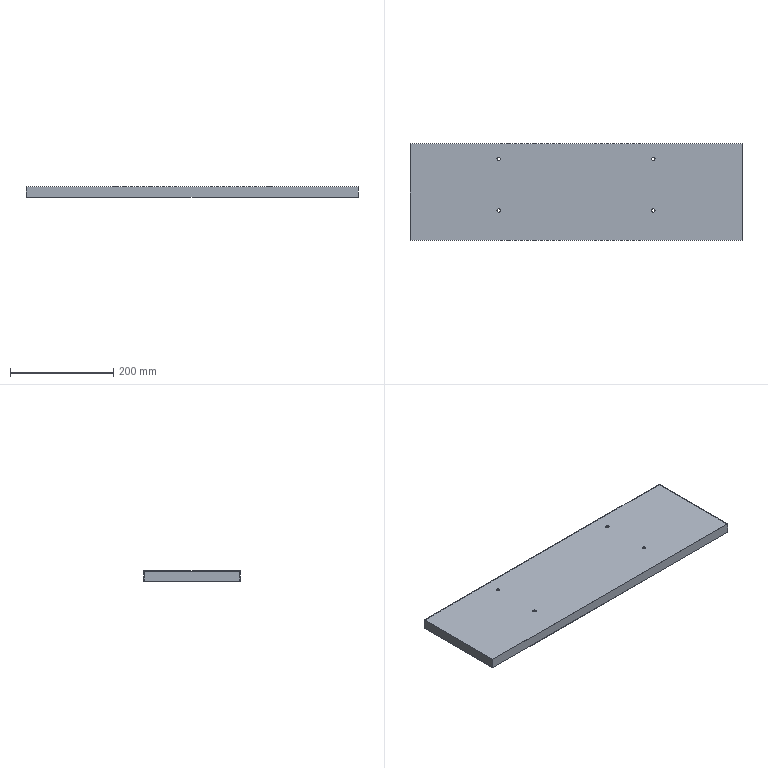Component | SolidWorks | FrameAssembly-1_FrameWeldment-1_FrontLowerThinPlate-1 | 1 solid | 19 faces | box 644 x 188 x 20 mm | volume 182559 mm3 | plane 11 | cylinder 8 | commonest cylinder face diameters 6.5 x8
build123d program:
from build123d import *

# Parameters (mm, degrees)
SKETCH1_W                      = 644
SKETCH1_H                      = 188
BOSS_EXTRUDE1_DEPTH            = 20
SKETCH2_W                      = 641.6
SKETCH2_H                      = 185.6
CUT_EXTRUDE1_DEPTH             = 18.8
F_6_5_6_5_DIAMETER_HOLE1_D     = 6.5
F_6_5_6_5_DIAMETER_HOLE1_DEPTH = 20


with BuildPart() as part:
    # Sketch1 → Boss-Extrude1 (new body)
    with BuildSketch(Plane(origin=(0, 0, 0), x_dir=(-1, 0, 0), z_dir=(0, 0, -1))):
        Rectangle(SKETCH1_W, SKETCH1_H)
    extrude(amount=-BOSS_EXTRUDE1_DEPTH)

    # Sketch2 → Cut-Extrude1 (cut)
    with BuildSketch(Plane(origin=(0, 0, 0), x_dir=(-1, 0, 0), z_dir=(0, 0, -1))):
        Rectangle(SKETCH2_W, SKETCH2_H)
    extrude(amount=-CUT_EXTRUDE1_DEPTH, mode=Mode.SUBTRACT)

    # 6.5 _6.5_ Diameter Hole1
    with Locations(Plane.XY.offset(20)):
        with Locations((-150, 64), (-150, -36), (150, 64), (150, -36)):
            Hole(F_6_5_6_5_DIAMETER_HOLE1_D / 2, depth=F_6_5_6_5_DIAMETER_HOLE1_DEPTH)


solid = part.part

# Placed as in the assembly
solid = solid.moved(Location((-298.746, -304.627, -36.5), (0, 0, 0)))
STEP:
#1=COLOUR_RGB('',0.7922,0.8196,0.9333);
#2=FILL_AREA_STYLE_COLOUR('',#1);
#3=FILL_AREA_STYLE('',(#2));
#4=SURFACE_STYLE_FILL_AREA(#3);
#5=SURFACE_SIDE_STYLE('',(#4));
#6=SURFACE_STYLE_USAGE(.BOTH.,#5);
#7=PRESENTATION_STYLE_ASSIGNMENT((#6));
#8=CARTESIAN_POINT('',(-17.539,-9.473,-0.6969));
#9=VERTEX_POINT('',#8);
#10=CARTESIAN_POINT('',(-17.795,-9.473,-0.6969));
#11=VERTEX_POINT('',#10);
#12=CARTESIAN_POINT('',(-17.667,-9.473,-0.6969));
#13=DIRECTION('',(0.,0.,-1.));
#14=DIRECTION('',(-1.,0.,0.));
#15=AXIS2_PLACEMENT_3D('',#12,#13,#14);
#16=CIRCLE('',#15,0.128);
#17=EDGE_CURVE('',#9,#11,#16,.T.);
#18=ORIENTED_EDGE('',*,*,#17,.T.);
#19=CARTESIAN_POINT('',(-17.795,-9.473,-0.6496));
#20=VERTEX_POINT('',#19);
#21=CARTESIAN_POINT('',(-17.795,-9.473,-0.6496));
#22=DIRECTION('',(0.,0.,1.));
#23=VECTOR('',#22,39.37);
#24=LINE('',#21,#23);
#25=EDGE_CURVE('',#11,#20,#24,.T.);
#26=ORIENTED_EDGE('',*,*,#25,.T.);
#27=CARTESIAN_POINT('',(-17.539,-9.473,-0.6496));
#28=VERTEX_POINT('',#27);
#29=CARTESIAN_POINT('',(-17.667,-9.473,-0.6496));
#30=DIRECTION('',(0.,0.,1.));
#31=DIRECTION('',(1.,0.,0.));
#32=AXIS2_PLACEMENT_3D('',#29,#30,#31);
#33=CIRCLE('',#32,0.128);
#34=EDGE_CURVE('',#20,#28,#33,.T.);
#35=ORIENTED_EDGE('',*,*,#34,.T.);
#36=CARTESIAN_POINT('',(-17.539,-9.473,-0.6496));
#37=DIRECTION('',(0.,0.,1.));
#38=VECTOR('',#37,39.37);
#39=LINE('',#36,#38);
#40=EDGE_CURVE('',#9,#28,#39,.T.);
#41=ORIENTED_EDGE('',*,*,#40,.F.);
#42=EDGE_LOOP('',(#18,#26,#35,#41));
#43=FACE_OUTER_BOUND('',#42,.T.);
#44=CARTESIAN_POINT('',(-17.667,-9.473,-0.6496));
#45=DIRECTION('',(0.,0.,1.));
#46=DIRECTION('',(1.,0.,0.));
#47=AXIS2_PLACEMENT_3D('',#44,#45,#46);
#48=CYLINDRICAL_SURFACE('',#47,0.128);
#49=ADVANCED_FACE('',(#43),#48,.F.);
#50=CARTESIAN_POINT('',(-17.539,-13.41,-0.6969));
#51=VERTEX_POINT('',#50);
#52=CARTESIAN_POINT('',(-17.795,-13.41,-0.6969));
#53=VERTEX_POINT('',#52);
#54=CARTESIAN_POINT('',(-17.667,-13.41,-0.6969));
#55=DIRECTION('',(0.,0.,-1.));
#56=DIRECTION('',(-1.,0.,0.));
#57=AXIS2_PLACEMENT_3D('',#54,#55,#56);
#58=CIRCLE('',#57,0.128);
#59=EDGE_CURVE('',#51,#53,#58,.T.);
#60=ORIENTED_EDGE('',*,*,#59,.T.);
#61=CARTESIAN_POINT('',(-17.795,-13.41,-0.6496));
#62=VERTEX_POINT('',#61);
#63=CARTESIAN_POINT('',(-17.795,-13.41,-0.6496));
#64=DIRECTION('',(0.,0.,1.));
#65=VECTOR('',#64,39.37);
#66=LINE('',#63,#65);
#67=EDGE_CURVE('',#53,#62,#66,.T.);
#68=ORIENTED_EDGE('',*,*,#67,.T.);
#69=CARTESIAN_POINT('',(-17.539,-13.41,-0.6496));
#70=VERTEX_POINT('',#69);
#71=CARTESIAN_POINT('',(-17.667,-13.41,-0.6496));
#72=DIRECTION('',(0.,0.,1.));
#73=DIRECTION('',(1.,0.,0.));
#74=AXIS2_PLACEMENT_3D('',#71,#72,#73);
#75=CIRCLE('',#74,0.128);
#76=EDGE_CURVE('',#62,#70,#75,.T.);
#77=ORIENTED_EDGE('',*,*,#76,.T.);
#78=CARTESIAN_POINT('',(-17.539,-13.41,-0.6496));
#79=DIRECTION('',(0.,0.,1.));
#80=VECTOR('',#79,39.37);
#81=LINE('',#78,#80);
#82=EDGE_CURVE('',#51,#70,#81,.T.);
#83=ORIENTED_EDGE('',*,*,#82,.F.);
#84=EDGE_LOOP('',(#60,#68,#77,#83));
#85=FACE_OUTER_BOUND('',#84,.T.);
#86=CARTESIAN_POINT('',(-17.667,-13.41,-0.6496));
#87=DIRECTION('',(0.,0.,1.));
#88=DIRECTION('',(1.,0.,0.));
#89=AXIS2_PLACEMENT_3D('',#86,#87,#88);
#90=CYLINDRICAL_SURFACE('',#89,0.128);
#91=ADVANCED_FACE('',(#85),#90,.F.);
#92=CARTESIAN_POINT('',(-5.728,-9.473,-0.6969));
#93=VERTEX_POINT('',#92);
#94=CARTESIAN_POINT('',(-5.984,-9.473,-0.6969));
#95=VERTEX_POINT('',#94);
#96=CARTESIAN_POINT('',(-5.856,-9.473,-0.6969));
#97=DIRECTION('',(0.,0.,-1.));
#98=DIRECTION('',(-1.,0.,0.));
#99=AXIS2_PLACEMENT_3D('',#96,#97,#98);
#100=CIRCLE('',#99,0.128);
#101=EDGE_CURVE('',#93,#95,#100,.T.);
#102=ORIENTED_EDGE('',*,*,#101,.T.);
#103=CARTESIAN_POINT('',(-5.984,-9.473,-0.6496));
#104=VERTEX_POINT('',#103);
#105=CARTESIAN_POINT('',(-5.984,-9.473,-0.6496));
#106=DIRECTION('',(0.,0.,1.));
#107=VECTOR('',#106,39.37);
#108=LINE('',#105,#107);
#109=EDGE_CURVE('',#95,#104,#108,.T.);
#110=ORIENTED_EDGE('',*,*,#109,.T.);
#111=CARTESIAN_POINT('',(-5.728,-9.473,-0.6496));
#112=VERTEX_POINT('',#111);
#113=CARTESIAN_POINT('',(-5.856,-9.473,-0.6496));
#114=DIRECTION('',(0.,0.,1.));
#115=DIRECTION('',(1.,0.,0.));
#116=AXIS2_PLACEMENT_3D('',#113,#114,#115);
#117=CIRCLE('',#116,0.128);
#118=EDGE_CURVE('',#104,#112,#117,.T.);
#119=ORIENTED_EDGE('',*,*,#118,.T.);
#120=CARTESIAN_POINT('',(-5.728,-9.473,-0.6496));
#121=DIRECTION('',(0.,0.,1.));
#122=VECTOR('',#121,39.37);
#123=LINE('',#120,#122);
#124=EDGE_CURVE('',#93,#112,#123,.T.);
#125=ORIENTED_EDGE('',*,*,#124,.F.);
#126=EDGE_LOOP('',(#102,#110,#119,#125));
#127=FACE_OUTER_BOUND('',#126,.T.);
#128=CARTESIAN_POINT('',(-5.856,-9.473,-0.6496));
#129=DIRECTION('',(0.,0.,1.));
#130=DIRECTION('',(1.,0.,0.));
#131=AXIS2_PLACEMENT_3D('',#128,#129,#130);
#132=CYLINDRICAL_SURFACE('',#131,0.128);
#133=ADVANCED_FACE('',(#127),#132,.F.);
#134=CARTESIAN_POINT('',(-5.728,-13.41,-0.6969));
#135=VERTEX_POINT('',#134);
#136=CARTESIAN_POINT('',(-5.984,-13.41,-0.6969));
#137=VERTEX_POINT('',#136);
#138=CARTESIAN_POINT('',(-5.856,-13.41,-0.6969));
#139=DIRECTION('',(0.,0.,-1.));
#140=DIRECTION('',(-1.,0.,0.));
#141=AXIS2_PLACEMENT_3D('',#138,#139,#140);
#142=CIRCLE('',#141,0.128);
#143=EDGE_CURVE('',#135,#137,#142,.T.);
#144=ORIENTED_EDGE('',*,*,#143,.T.);
#145=CARTESIAN_POINT('',(-5.984,-13.41,-0.6496));
#146=VERTEX_POINT('',#145);
#147=CARTESIAN_POINT('',(-5.984,-13.41,-0.6496));
#148=DIRECTION('',(0.,0.,1.));
#149=VECTOR('',#148,39.37);
#150=LINE('',#147,#149);
#151=EDGE_CURVE('',#137,#146,#150,.T.);
#152=ORIENTED_EDGE('',*,*,#151,.T.);
#153=CARTESIAN_POINT('',(-5.728,-13.41,-0.6496));
#154=VERTEX_POINT('',#153);
#155=CARTESIAN_POINT('',(-5.856,-13.41,-0.6496));
#156=DIRECTION('',(0.,0.,1.));
#157=DIRECTION('',(1.,0.,0.));
#158=AXIS2_PLACEMENT_3D('',#155,#156,#157);
#159=CIRCLE('',#158,0.128);
#160=EDGE_CURVE('',#146,#154,#159,.T.);
#161=ORIENTED_EDGE('',*,*,#160,.T.);
#162=CARTESIAN_POINT('',(-5.728,-13.41,-0.6496));
#163=DIRECTION('',(0.,0.,1.));
#164=VECTOR('',#163,39.37);
#165=LINE('',#162,#164);
#166=EDGE_CURVE('',#135,#154,#165,.T.);
#167=ORIENTED_EDGE('',*,*,#166,.F.);
#168=EDGE_LOOP('',(#144,#152,#161,#167));
#169=FACE_OUTER_BOUND('',#168,.T.);
#170=CARTESIAN_POINT('',(-5.856,-13.41,-0.6496));
#171=DIRECTION('',(0.,0.,1.));
#172=DIRECTION('',(1.,0.,0.));
#173=AXIS2_PLACEMENT_3D('',#170,#171,#172);
#174=CYLINDRICAL_SURFACE('',#173,0.128);
#175=ADVANCED_FACE('',(#169),#174,.F.);
#176=CARTESIAN_POINT('',(0.9155,-15.694,-1.437));
#177=VERTEX_POINT('',#176);
#178=CARTESIAN_POINT('',(-24.439,-15.694,-1.437));
#179=VERTEX_POINT('',#178);
#180=CARTESIAN_POINT('',(0.9155,-15.694,-1.437));
#181=DIRECTION('',(-1.,0.,0.));
#182=VECTOR('',#181,39.37);
#183=LINE('',#180,#182);
#184=EDGE_CURVE('',#177,#179,#183,.T.);
#185=ORIENTED_EDGE('',*,*,#184,.F.);
#186=CARTESIAN_POINT('',(0.9155,-15.694,-0.6496));
#187=VERTEX_POINT('',#186);
#188=CARTESIAN_POINT('',(0.9155,-15.694,-0.6496));
#189=DIRECTION('',(0.,0.,-1.));
#190=VECTOR('',#189,39.37);
#191=LINE('',#188,#190);
#192=EDGE_CURVE('',#187,#177,#191,.T.);
#193=ORIENTED_EDGE('',*,*,#192,.F.);
#194=CARTESIAN_POINT('',(-24.439,-15.694,-0.6496));
#195=VERTEX_POINT('',#194);
#196=CARTESIAN_POINT('',(0.9155,-15.694,-0.6496));
#197=DIRECTION('',(-1.,0.,0.));
#198=VECTOR('',#197,39.37);
#199=LINE('',#196,#198);
#200=EDGE_CURVE('',#187,#195,#199,.T.);
#201=ORIENTED_EDGE('',*,*,#200,.T.);
#202=CARTESIAN_POINT('',(-24.439,-15.694,-0.6496));
#203=DIRECTION('',(0.,0.,-1.));
#204=VECTOR('',#203,39.37);
#205=LINE('',#202,#204);
#206=EDGE_CURVE('',#195,#179,#205,.T.);
#207=ORIENTED_EDGE('',*,*,#206,.T.);
#208=EDGE_LOOP('',(#185,#193,#201,#207));
#209=FACE_OUTER_BOUND('',#208,.T.);
#210=CARTESIAN_POINT('',(0.9155,-15.694,-0.6496));
#211=DIRECTION('',(0.,-1.,0.));
#212=DIRECTION('',(0.,0.,-1.));
#213=AXIS2_PLACEMENT_3D('',#210,#211,#212);
#214=PLANE('',#213);
#215=ADVANCED_FACE('',(#209),#214,.T.);
#216=CARTESIAN_POINT('',(0.9155,-8.292,-1.437));
#217=VERTEX_POINT('',#216);
#218=CARTESIAN_POINT('',(0.9155,-8.292,-1.437));
#219=DIRECTION('',(-0.,-1.,0.));
#220=VECTOR('',#219,39.37);
#221=LINE('',#218,#220);
#222=EDGE_CURVE('',#217,#177,#221,.T.);
#223=ORIENTED_EDGE('',*,*,#222,.F.);
#224=CARTESIAN_POINT('',(0.9155,-8.292,-0.6496));
#225=VERTEX_POINT('',#224);
#226=CARTESIAN_POINT('',(0.9155,-8.292,-0.6496));
#227=DIRECTION('',(0.,0.,-1.));
#228=VECTOR('',#227,39.37);
#229=LINE('',#226,#228);
#230=EDGE_CURVE('',#225,#217,#229,.T.);
#231=ORIENTED_EDGE('',*,*,#230,.F.);
#232=CARTESIAN_POINT('',(0.9155,-8.292,-0.6496));
#233=DIRECTION('',(-0.,-1.,0.));
#234=VECTOR('',#233,39.37);
#235=LINE('',#232,#234);
#236=EDGE_CURVE('',#225,#187,#235,.T.);
#237=ORIENTED_EDGE('',*,*,#236,.T.);
#238=ORIENTED_EDGE('',*,*,#192,.T.);
#239=EDGE_LOOP('',(#223,#231,#237,#238));
#240=FACE_OUTER_BOUND('',#239,.T.);
#241=CARTESIAN_POINT('',(0.9155,-8.292,-0.6496));
#242=DIRECTION('',(1.,-0.,0.));
#243=DIRECTION('',(0.,1.,0.));
#244=AXIS2_PLACEMENT_3D('',#241,#242,#243);
#245=PLANE('',#244);
#246=ADVANCED_FACE('',(#240),#245,.T.);
#247=CARTESIAN_POINT('',(-24.439,-8.292,-1.437));
#248=VERTEX_POINT('',#247);
#249=CARTESIAN_POINT('',(-24.439,-8.292,-1.437));
#250=DIRECTION('',(1.,0.,0.));
#251=VECTOR('',#250,39.37);
#252=LINE('',#249,#251);
#253=EDGE_CURVE('',#248,#217,#252,.T.);
#254=ORIENTED_EDGE('',*,*,#253,.F.);
#255=CARTESIAN_POINT('',(-24.439,-8.292,-0.6496));
#256=VERTEX_POINT('',#255);
#257=CARTESIAN_POINT('',(-24.439,-8.292,-0.6496));
#258=DIRECTION('',(0.,0.,-1.));
#259=VECTOR('',#258,39.37);
#260=LINE('',#257,#259);
#261=EDGE_CURVE('',#256,#248,#260,.T.);
#262=ORIENTED_EDGE('',*,*,#261,.F.);
#263=CARTESIAN_POINT('',(-24.439,-8.292,-0.6496));
#264=DIRECTION('',(1.,0.,0.));
#265=VECTOR('',#264,39.37);
#266=LINE('',#263,#265);
#267=EDGE_CURVE('',#256,#225,#266,.T.);
#268=ORIENTED_EDGE('',*,*,#267,.T.);
#269=ORIENTED_EDGE('',*,*,#230,.T.);
#270=EDGE_LOOP('',(#254,#262,#268,#269));
#271=FACE_OUTER_BOUND('',#270,.T.);
#272=CARTESIAN_POINT('',(-24.439,-8.292,-0.6496));
#273=DIRECTION('',(0.,1.,0.));
#274=DIRECTION('',(0.,0.,1.));
#275=AXIS2_PLACEMENT_3D('',#272,#273,#274);
#276=PLANE('',#275);
#277=ADVANCED_FACE('',(#271),#276,.T.);
#278=CARTESIAN_POINT('',(-24.439,-15.694,-1.437));
#279=DIRECTION('',(0.,1.,0.));
#280=VECTOR('',#279,39.37);
#281=LINE('',#278,#280);
#282=EDGE_CURVE('',#179,#248,#281,.T.);
#283=ORIENTED_EDGE('',*,*,#282,.F.);
#284=ORIENTED_EDGE('',*,*,#206,.F.);
#285=CARTESIAN_POINT('',(-24.439,-15.694,-0.6496));
#286=DIRECTION('',(0.,1.,0.));
#287=VECTOR('',#286,39.37);
#288=LINE('',#285,#287);
#289=EDGE_CURVE('',#195,#256,#288,.T.);
#290=ORIENTED_EDGE('',*,*,#289,.T.);
#291=ORIENTED_EDGE('',*,*,#261,.T.);
#292=EDGE_LOOP('',(#283,#284,#290,#291));
#293=FACE_OUTER_BOUND('',#292,.T.);
#294=CARTESIAN_POINT('',(-24.439,-15.694,-0.6496));
#295=DIRECTION('',(-1.,0.,0.));
#296=DIRECTION('',(0.,0.,1.));
#297=AXIS2_PLACEMENT_3D('',#294,#295,#296);
#298=PLANE('',#297);
#299=ADVANCED_FACE('',(#293),#298,.T.);
#300=CARTESIAN_POINT('',(-17.667,-9.473,-0.6496));
#301=DIRECTION('',(0.,0.,1.));
#302=DIRECTION('',(1.,0.,0.));
#303=AXIS2_PLACEMENT_3D('',#300,#301,#302);
#304=CIRCLE('',#303,0.128);
#305=EDGE_CURVE('',#28,#20,#304,.T.);
#306=ORIENTED_EDGE('',*,*,#305,.F.);
#307=ORIENTED_EDGE('',*,*,#34,.F.);
#308=EDGE_LOOP('',(#306,#307));
#309=FACE_BOUND('',#308,.T.);
#310=CARTESIAN_POINT('',(-17.667,-13.41,-0.6496));
#311=DIRECTION('',(0.,0.,1.));
#312=DIRECTION('',(1.,0.,0.));
#313=AXIS2_PLACEMENT_3D('',#310,#311,#312);
#314=CIRCLE('',#313,0.128);
#315=EDGE_CURVE('',#70,#62,#314,.T.);
#316=ORIENTED_EDGE('',*,*,#315,.F.);
#317=ORIENTED_EDGE('',*,*,#76,.F.);
#318=EDGE_LOOP('',(#316,#317));
#319=FACE_BOUND('',#318,.T.);
#320=CARTESIAN_POINT('',(-5.856,-9.473,-0.6496));
#321=DIRECTION('',(0.,0.,1.));
#322=DIRECTION('',(1.,0.,0.));
#323=AXIS2_PLACEMENT_3D('',#320,#321,#322);
#324=CIRCLE('',#323,0.128);
#325=EDGE_CURVE('',#112,#104,#324,.T.);
#326=ORIENTED_EDGE('',*,*,#325,.F.);
#327=ORIENTED_EDGE('',*,*,#118,.F.);
#328=EDGE_LOOP('',(#326,#327));
#329=FACE_BOUND('',#328,.T.);
#330=CARTESIAN_POINT('',(-5.856,-13.41,-0.6496));
#331=DIRECTION('',(0.,0.,1.));
#332=DIRECTION('',(1.,0.,0.));
#333=AXIS2_PLACEMENT_3D('',#330,#331,#332);
#334=CIRCLE('',#333,0.128);
#335=EDGE_CURVE('',#154,#146,#334,.T.);
#336=ORIENTED_EDGE('',*,*,#335,.F.);
#337=ORIENTED_EDGE('',*,*,#160,.F.);
#338=EDGE_LOOP('',(#336,#337));
#339=FACE_BOUND('',#338,.T.);
#340=ORIENTED_EDGE('',*,*,#200,.F.);
#341=ORIENTED_EDGE('',*,*,#236,.F.);
#342=ORIENTED_EDGE('',*,*,#267,.F.);
#343=ORIENTED_EDGE('',*,*,#289,.F.);
#344=EDGE_LOOP('',(#340,#341,#342,#343));
#345=FACE_OUTER_BOUND('',#344,.T.);
#346=CARTESIAN_POINT('',(-11.762,-11.993,-0.6496));
#347=DIRECTION('',(0.,0.,-1.));
#348=DIRECTION('',(-1.,0.,0.));
#349=AXIS2_PLACEMENT_3D('',#346,#347,#348);
#350=PLANE('',#349);
#351=ADVANCED_FACE('',(#309,#319,#329,#339,#345),#350,.F.);
#352=CARTESIAN_POINT('',(0.8683,-8.34,-1.437));
#353=VERTEX_POINT('',#352);
#354=CARTESIAN_POINT('',(0.8683,-15.647,-1.437));
#355=VERTEX_POINT('',#354);
#356=CARTESIAN_POINT('',(0.8683,-8.34,-1.437));
#357=DIRECTION('',(0.,-1.,0.));
#358=VECTOR('',#357,39.37);
#359=LINE('',#356,#358);
#360=EDGE_CURVE('',#353,#355,#359,.T.);
#361=ORIENTED_EDGE('',*,*,#360,.F.);
#362=CARTESIAN_POINT('',(-24.392,-8.34,-1.437));
#363=VERTEX_POINT('',#362);
#364=CARTESIAN_POINT('',(-24.392,-8.34,-1.437));
#365=DIRECTION('',(1.,0.,0.));
#366=VECTOR('',#365,39.37);
#367=LINE('',#364,#366);
#368=EDGE_CURVE('',#363,#353,#367,.T.);
#369=ORIENTED_EDGE('',*,*,#368,.F.);
#370=CARTESIAN_POINT('',(-24.392,-15.647,-1.437));
#371=VERTEX_POINT('',#370);
#372=CARTESIAN_POINT('',(-24.392,-15.647,-1.437));
#373=DIRECTION('',(0.,1.,0.));
#374=VECTOR('',#373,39.37);
#375=LINE('',#372,#374);
#376=EDGE_CURVE('',#371,#363,#375,.T.);
#377=ORIENTED_EDGE('',*,*,#376,.F.);
#378=CARTESIAN_POINT('',(0.8683,-15.647,-1.437));
#379=DIRECTION('',(-1.,0.,0.));
#380=VECTOR('',#379,39.37);
#381=LINE('',#378,#380);
#382=EDGE_CURVE('',#355,#371,#381,.T.);
#383=ORIENTED_EDGE('',*,*,#382,.F.);
#384=EDGE_LOOP('',(#361,#369,#377,#383));
#385=FACE_BOUND('',#384,.T.);
#386=ORIENTED_EDGE('',*,*,#184,.T.);
#387=ORIENTED_EDGE('',*,*,#282,.T.);
#388=ORIENTED_EDGE('',*,*,#253,.T.);
#389=ORIENTED_EDGE('',*,*,#222,.T.);
#390=EDGE_LOOP('',(#386,#387,#388,#389));
#391=FACE_OUTER_BOUND('',#390,.T.);
#392=CARTESIAN_POINT('',(-11.762,-11.993,-1.437));
#393=DIRECTION('',(0.,0.,-1.));
#394=DIRECTION('',(-1.,0.,0.));
#395=AXIS2_PLACEMENT_3D('',#392,#393,#394);
#396=PLANE('',#395);
#397=ADVANCED_FACE('',(#385,#391),#396,.T.);
#398=ORIENTED_EDGE('',*,*,#360,.T.);
#399=CARTESIAN_POINT('',(0.8683,-15.647,-0.6969));
#400=VERTEX_POINT('',#399);
#401=CARTESIAN_POINT('',(0.8683,-15.647,-0.6969));
#402=DIRECTION('',(0.,0.,-1.));
#403=VECTOR('',#402,39.37);
#404=LINE('',#401,#403);
#405=EDGE_CURVE('',#400,#355,#404,.T.);
#406=ORIENTED_EDGE('',*,*,#405,.F.);
#407=CARTESIAN_POINT('',(0.8683,-8.34,-0.6969));
#408=VERTEX_POINT('',#407);
#409=CARTESIAN_POINT('',(0.8683,-8.34,-0.6969));
#410=DIRECTION('',(0.,-1.,0.));
#411=VECTOR('',#410,39.37);
#412=LINE('',#409,#411);
#413=EDGE_CURVE('',#408,#400,#412,.T.);
#414=ORIENTED_EDGE('',*,*,#413,.F.);
#415=CARTESIAN_POINT('',(0.8683,-8.34,-0.6969));
#416=DIRECTION('',(0.,0.,-1.));
#417=VECTOR('',#416,39.37);
#418=LINE('',#415,#417);
#419=EDGE_CURVE('',#408,#353,#418,.T.);
#420=ORIENTED_EDGE('',*,*,#419,.T.);
#421=EDGE_LOOP('',(#398,#406,#414,#420));
#422=FACE_OUTER_BOUND('',#421,.T.);
#423=CARTESIAN_POINT('',(0.8683,-8.34,-0.6969));
#424=DIRECTION('',(1.,0.,0.));
#425=DIRECTION('',(0.,0.,-1.));
#426=AXIS2_PLACEMENT_3D('',#423,#424,#425);
#427=PLANE('',#426);
#428=ADVANCED_FACE('',(#422),#427,.F.);
#429=ORIENTED_EDGE('',*,*,#368,.T.);
#430=ORIENTED_EDGE('',*,*,#419,.F.);
#431=CARTESIAN_POINT('',(-24.392,-8.34,-0.6969));
#432=VERTEX_POINT('',#431);
#433=CARTESIAN_POINT('',(-24.392,-8.34,-0.6969));
#434=DIRECTION('',(1.,0.,0.));
#435=VECTOR('',#434,39.37);
#436=LINE('',#433,#435);
#437=EDGE_CURVE('',#432,#408,#436,.T.);
#438=ORIENTED_EDGE('',*,*,#437,.F.);
#439=CARTESIAN_POINT('',(-24.392,-8.34,-0.6969));
#440=DIRECTION('',(0.,0.,-1.));
#441=VECTOR('',#440,39.37);
#442=LINE('',#439,#441);
#443=EDGE_CURVE('',#432,#363,#442,.T.);
#444=ORIENTED_EDGE('',*,*,#443,.T.);
#445=EDGE_LOOP('',(#429,#430,#438,#444));
#446=FACE_OUTER_BOUND('',#445,.T.);
#447=CARTESIAN_POINT('',(-24.392,-8.34,-0.6969));
#448=DIRECTION('',(0.,1.,0.));
#449=DIRECTION('',(0.,0.,1.));
#450=AXIS2_PLACEMENT_3D('',#447,#448,#449);
#451=PLANE('',#450);
#452=ADVANCED_FACE('',(#446),#451,.F.);
#453=ORIENTED_EDGE('',*,*,#376,.T.);
#454=ORIENTED_EDGE('',*,*,#443,.F.);
#455=CARTESIAN_POINT('',(-24.392,-15.647,-0.6969));
#456=VERTEX_POINT('',#455);
#457=CARTESIAN_POINT('',(-24.392,-15.647,-0.6969));
#458=DIRECTION('',(0.,1.,0.));
#459=VECTOR('',#458,39.37);
#460=LINE('',#457,#459);
#461=EDGE_CURVE('',#456,#432,#460,.T.);
#462=ORIENTED_EDGE('',*,*,#461,.F.);
#463=CARTESIAN_POINT('',(-24.392,-15.647,-0.6969));
#464=DIRECTION('',(0.,0.,-1.));
#465=VECTOR('',#464,39.37);
#466=LINE('',#463,#465);
#467=EDGE_CURVE('',#456,#371,#466,.T.);
#468=ORIENTED_EDGE('',*,*,#467,.T.);
#469=EDGE_LOOP('',(#453,#454,#462,#468));
#470=FACE_OUTER_BOUND('',#469,.T.);
#471=CARTESIAN_POINT('',(-24.392,-15.647,-0.6969));
#472=DIRECTION('',(-1.,0.,0.));
#473=DIRECTION('',(0.,0.,1.));
#474=AXIS2_PLACEMENT_3D('',#471,#472,#473);
#475=PLANE('',#474);
#476=ADVANCED_FACE('',(#470),#475,.F.);
#477=ORIENTED_EDGE('',*,*,#382,.T.);
#478=ORIENTED_EDGE('',*,*,#467,.F.);
#479=CARTESIAN_POINT('',(0.8683,-15.647,-0.6969));
#480=DIRECTION('',(-1.,0.,0.));
#481=VECTOR('',#480,39.37);
#482=LINE('',#479,#481);
#483=EDGE_CURVE('',#400,#456,#482,.T.);
#484=ORIENTED_EDGE('',*,*,#483,.F.);
#485=ORIENTED_EDGE('',*,*,#405,.T.);
#486=EDGE_LOOP('',(#477,#478,#484,#485));
#487=FACE_OUTER_BOUND('',#486,.T.);
#488=CARTESIAN_POINT('',(0.8683,-15.647,-0.6969));
#489=DIRECTION('',(0.,-1.,0.));
#490=DIRECTION('',(0.,0.,-1.));
#491=AXIS2_PLACEMENT_3D('',#488,#489,#490);
#492=PLANE('',#491);
#493=ADVANCED_FACE('',(#487),#492,.F.);
#494=ORIENTED_EDGE('',*,*,#17,.F.);
#495=CARTESIAN_POINT('',(-17.667,-9.473,-0.6969));
#496=DIRECTION('',(0.,0.,-1.));
#497=DIRECTION('',(-1.,0.,0.));
#498=AXIS2_PLACEMENT_3D('',#495,#496,#497);
#499=CIRCLE('',#498,0.128);
#500=EDGE_CURVE('',#11,#9,#499,.T.);
#501=ORIENTED_EDGE('',*,*,#500,.F.);
#502=EDGE_LOOP('',(#494,#501));
#503=FACE_BOUND('',#502,.T.);
#504=ORIENTED_EDGE('',*,*,#59,.F.);
#505=CARTESIAN_POINT('',(-17.667,-13.41,-0.6969));
#506=DIRECTION('',(0.,0.,-1.));
#507=DIRECTION('',(-1.,0.,0.));
#508=AXIS2_PLACEMENT_3D('',#505,#506,#507);
#509=CIRCLE('',#508,0.128);
#510=EDGE_CURVE('',#53,#51,#509,.T.);
#511=ORIENTED_EDGE('',*,*,#510,.F.);
#512=EDGE_LOOP('',(#504,#511));
#513=FACE_BOUND('',#512,.T.);
#514=ORIENTED_EDGE('',*,*,#101,.F.);
#515=CARTESIAN_POINT('',(-5.856,-9.473,-0.6969));
#516=DIRECTION('',(0.,0.,-1.));
#517=DIRECTION('',(-1.,0.,0.));
#518=AXIS2_PLACEMENT_3D('',#515,#516,#517);
#519=CIRCLE('',#518,0.128);
#520=EDGE_CURVE('',#95,#93,#519,.T.);
#521=ORIENTED_EDGE('',*,*,#520,.F.);
#522=EDGE_LOOP('',(#514,#521));
#523=FACE_BOUND('',#522,.T.);
#524=ORIENTED_EDGE('',*,*,#143,.F.);
#525=CARTESIAN_POINT('',(-5.856,-13.41,-0.6969));
#526=DIRECTION('',(0.,0.,-1.));
#527=DIRECTION('',(-1.,0.,0.));
#528=AXIS2_PLACEMENT_3D('',#525,#526,#527);
#529=CIRCLE('',#528,0.128);
#530=EDGE_CURVE('',#137,#135,#529,.T.);
#531=ORIENTED_EDGE('',*,*,#530,.F.);
#532=EDGE_LOOP('',(#524,#531));
#533=FACE_BOUND('',#532,.T.);
#534=ORIENTED_EDGE('',*,*,#413,.T.);
#535=ORIENTED_EDGE('',*,*,#483,.T.);
#536=ORIENTED_EDGE('',*,*,#461,.T.);
#537=ORIENTED_EDGE('',*,*,#437,.T.);
#538=EDGE_LOOP('',(#534,#535,#536,#537));
#539=FACE_OUTER_BOUND('',#538,.T.);
#540=CARTESIAN_POINT('',(-11.762,-11.993,-0.6969));
#541=DIRECTION('',(0.,0.,-1.));
#542=DIRECTION('',(-1.,0.,0.));
#543=AXIS2_PLACEMENT_3D('',#540,#541,#542);
#544=PLANE('',#543);
#545=ADVANCED_FACE('',(#503,#513,#523,#533,#539),#544,.T.);
#546=ORIENTED_EDGE('',*,*,#151,.F.);
#547=ORIENTED_EDGE('',*,*,#530,.T.);
#548=ORIENTED_EDGE('',*,*,#166,.T.);
#549=ORIENTED_EDGE('',*,*,#335,.T.);
#550=EDGE_LOOP('',(#546,#547,#548,#549));
#551=FACE_OUTER_BOUND('',#550,.T.);
#552=CARTESIAN_POINT('',(-5.856,-13.41,-0.6496));
#553=DIRECTION('',(0.,0.,1.));
#554=DIRECTION('',(1.,0.,0.));
#555=AXIS2_PLACEMENT_3D('',#552,#553,#554);
#556=CYLINDRICAL_SURFACE('',#555,0.128);
#557=ADVANCED_FACE('',(#551),#556,.F.);
#558=ORIENTED_EDGE('',*,*,#109,.F.);
#559=ORIENTED_EDGE('',*,*,#520,.T.);
#560=ORIENTED_EDGE('',*,*,#124,.T.);
#561=ORIENTED_EDGE('',*,*,#325,.T.);
#562=EDGE_LOOP('',(#558,#559,#560,#561));
#563=FACE_OUTER_BOUND('',#562,.T.);
#564=CARTESIAN_POINT('',(-5.856,-9.473,-0.6496));
#565=DIRECTION('',(0.,0.,1.));
#566=DIRECTION('',(1.,0.,0.));
#567=AXIS2_PLACEMENT_3D('',#564,#565,#566);
#568=CYLINDRICAL_SURFACE('',#567,0.128);
#569=ADVANCED_FACE('',(#563),#568,.F.);
#570=ORIENTED_EDGE('',*,*,#67,.F.);
#571=ORIENTED_EDGE('',*,*,#510,.T.);
#572=ORIENTED_EDGE('',*,*,#82,.T.);
#573=ORIENTED_EDGE('',*,*,#315,.T.);
#574=EDGE_LOOP('',(#570,#571,#572,#573));
#575=FACE_OUTER_BOUND('',#574,.T.);
#576=CARTESIAN_POINT('',(-17.667,-13.41,-0.6496));
#577=DIRECTION('',(0.,0.,1.));
#578=DIRECTION('',(1.,0.,0.));
#579=AXIS2_PLACEMENT_3D('',#576,#577,#578);
#580=CYLINDRICAL_SURFACE('',#579,0.128);
#581=ADVANCED_FACE('',(#575),#580,.F.);
#582=ORIENTED_EDGE('',*,*,#25,.F.);
#583=ORIENTED_EDGE('',*,*,#500,.T.);
#584=ORIENTED_EDGE('',*,*,#40,.T.);
#585=ORIENTED_EDGE('',*,*,#305,.T.);
#586=EDGE_LOOP('',(#582,#583,#584,#585));
#587=FACE_OUTER_BOUND('',#586,.T.);
#588=CARTESIAN_POINT('',(-17.667,-9.473,-0.6496));
#589=DIRECTION('',(0.,0.,1.));
#590=DIRECTION('',(1.,0.,0.));
#591=AXIS2_PLACEMENT_3D('',#588,#589,#590);
#592=CYLINDRICAL_SURFACE('',#591,0.128);
#593=ADVANCED_FACE('',(#587),#592,.F.);
#594=CLOSED_SHELL('',(#49,#91,#133,#175,#215,#246,#277,#299,#351,#397,#428,#452,#476,#493,#545,#557,#569,#581,#593));
#595=MANIFOLD_SOLID_BREP('',#594);
#596=STYLED_ITEM('',(#7),#595);
#597=(LENGTH_UNIT()NAMED_UNIT(*)SI_UNIT($,.METRE.));
#598=LENGTH_MEASURE_WITH_UNIT(LENGTH_MEASURE(0.0254),#597);
#599=DIMENSIONAL_EXPONENTS(1.,0.,0.,0.,0.,0.,0.);
#600=(CONVERSION_BASED_UNIT('',#598)LENGTH_UNIT()NAMED_UNIT(#599));
#601=UNCERTAINTY_MEASURE_WITH_UNIT(LENGTH_MEASURE(0.00001),#600,'','');
#602=(NAMED_UNIT(*)PLANE_ANGLE_UNIT()SI_UNIT($,.RADIAN.));
#603=(NAMED_UNIT(*)SI_UNIT($,.STERADIAN.)SOLID_ANGLE_UNIT());
#604=(GEOMETRIC_REPRESENTATION_CONTEXT(3)GLOBAL_UNCERTAINTY_ASSIGNED_CONTEXT((#601))GLOBAL_UNIT_ASSIGNED_CONTEXT((#600,#602,#603))REPRESENTATION_CONTEXT('',''));
#605=MECHANICAL_DESIGN_GEOMETRIC_PRESENTATION_REPRESENTATION('',(#596),#604);
#606=PRESENTATION_LAYER_ASSIGNMENT('','',(#596));
#607=CARTESIAN_POINT('',(0.,0.,0.));
#608=DIRECTION('',(0.,0.,1.));
#609=DIRECTION('',(1.,0.,0.));
#610=AXIS2_PLACEMENT_3D('',#607,#608,#609);
#611=(LENGTH_UNIT()NAMED_UNIT(*)SI_UNIT($,.METRE.));
#612=LENGTH_MEASURE_WITH_UNIT(LENGTH_MEASURE(0.0254),#611);
#613=DIMENSIONAL_EXPONENTS(1.,0.,0.,0.,0.,0.,0.);
#614=(CONVERSION_BASED_UNIT('',#612)LENGTH_UNIT()NAMED_UNIT(#613));
#615=UNCERTAINTY_MEASURE_WITH_UNIT(LENGTH_MEASURE(0.00001),#614,'','');
#616=(NAMED_UNIT(*)PLANE_ANGLE_UNIT()SI_UNIT($,.RADIAN.));
#617=(NAMED_UNIT(*)SI_UNIT($,.STERADIAN.)SOLID_ANGLE_UNIT());
#618=(GEOMETRIC_REPRESENTATION_CONTEXT(3)GLOBAL_UNCERTAINTY_ASSIGNED_CONTEXT((#615))GLOBAL_UNIT_ASSIGNED_CONTEXT((#614,#616,#617))REPRESENTATION_CONTEXT('',''));
#619=ADVANCED_BREP_SHAPE_REPRESENTATION('',(#595,#610),#618);